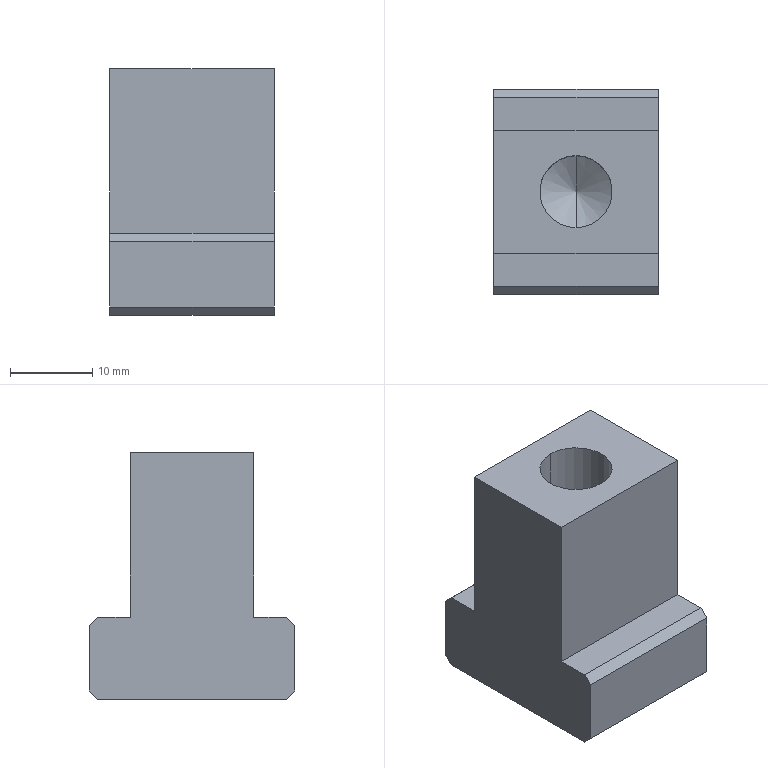Component | SolidWorks | 19-1 | 1 solid | 18 faces | box 20 x 25 x 30 mm | volume 9386 mm3 | plane 14 | cylinder 2 | cone 2 | commonest cylinder face diameters 8.8 x2
build123d program:
from build123d import *

# Parameters (mm, degrees)
SKETCH1_W                   = 20
SKETCH1_H                   = 25
EXTRUDE1_DEPTH              = 10
SKETCH2_W                   = 20
SKETCH2_H                   = 15
EXTRUDE2_DEPTH              = 20
M10X1_25_TAPPED_HOLE1_D     = 8.8
M10X1_25_TAPPED_HOLE1_DEPTH = 25
M10X1_25_TAPPED_HOLE1_TIP   = 2.644
CHAMFER1_SIZE               = 1


with BuildPart() as part:
    # Sketch1 → Extrude1 (new body)
    with BuildSketch(Plane(origin=(0, 0, 0), x_dir=(1, 0, 0), z_dir=(0, 1, 0))):
        Rectangle(SKETCH1_W, SKETCH1_H)
    extrude(amount=EXTRUDE1_DEPTH)

    # Sketch2 → Extrude2 (add)
    with BuildSketch(Plane(origin=(0, 10, 0), x_dir=(1, 0, 0), z_dir=(0, 1, 0))):
        Rectangle(SKETCH2_W, SKETCH2_H)
    extrude(amount=EXTRUDE2_DEPTH)

    # M10x1.25 Tapped Hole1
    with Locations(Plane(origin=(0, 30, 0), x_dir=(1, 0, 0), z_dir=(0, 1, 0))):
        with Locations((0, 0)):
            Hole(M10X1_25_TAPPED_HOLE1_D / 2, depth=M10X1_25_TAPPED_HOLE1_DEPTH)
            with Locations((0, 0, -(M10X1_25_TAPPED_HOLE1_DEPTH + M10X1_25_TAPPED_HOLE1_TIP / 2))):  # 118° drill point
                Cone(0, M10X1_25_TAPPED_HOLE1_D / 2, M10X1_25_TAPPED_HOLE1_TIP, mode=Mode.SUBTRACT)

    # Chamfer1
    chamfer1_edges = [part.edges().sort_by_distance(p)[0] for p in [
        (0, 10, -12.5),
        (0, 0, -12.5),
        (0, 10, 12.5),
        (0, 0, 12.5),
    ]]
    chamfer(chamfer1_edges, length=CHAMFER1_SIZE)


solid = part.part

# Placed as in the assembly
solid = solid.moved(Location((-102.5, -29.5, 100.8), (90, 0, 0)))
STEP:
#1=COLOUR_RGB('',0.7922,0.8196,0.9333);
#2=FILL_AREA_STYLE_COLOUR('',#1);
#3=FILL_AREA_STYLE('',(#2));
#4=SURFACE_STYLE_FILL_AREA(#3);
#5=SURFACE_SIDE_STYLE('',(#4));
#6=SURFACE_STYLE_USAGE(.BOTH.,#5);
#7=PRESENTATION_STYLE_ASSIGNMENT((#6));
#8=CARTESIAN_POINT('',(-4.035,-0.9882,4.165));
#9=VERTEX_POINT('',#8);
#10=CARTESIAN_POINT('',(-4.035,-1.335,4.165));
#11=VERTEX_POINT('',#10);
#12=CARTESIAN_POINT('',(-4.035,-1.161,4.165));
#13=DIRECTION('',(0.,0.,1.));
#14=DIRECTION('',(0.,-1.,0.));
#15=AXIS2_PLACEMENT_3D('',#12,#13,#14);
#16=CIRCLE('',#15,0.1732);
#17=EDGE_CURVE('',#9,#11,#16,.T.);
#18=ORIENTED_EDGE('',*,*,#17,.F.);
#19=CARTESIAN_POINT('',(-4.035,-0.9882,5.15));
#20=VERTEX_POINT('',#19);
#21=CARTESIAN_POINT('',(-4.035,-0.9882,5.15));
#22=DIRECTION('',(0.,0.,1.));
#23=VECTOR('',#22,39.37);
#24=LINE('',#21,#23);
#25=EDGE_CURVE('',#9,#20,#24,.T.);
#26=ORIENTED_EDGE('',*,*,#25,.T.);
#27=CARTESIAN_POINT('',(-4.035,-1.335,5.15));
#28=VERTEX_POINT('',#27);
#29=CARTESIAN_POINT('',(-4.035,-1.161,5.15));
#30=DIRECTION('',(0.,0.,1.));
#31=DIRECTION('',(0.,-1.,0.));
#32=AXIS2_PLACEMENT_3D('',#29,#30,#31);
#33=CIRCLE('',#32,0.1732);
#34=EDGE_CURVE('',#20,#28,#33,.T.);
#35=ORIENTED_EDGE('',*,*,#34,.T.);
#36=CARTESIAN_POINT('',(-4.035,-1.335,5.15));
#37=DIRECTION('',(0.,0.,1.));
#38=VECTOR('',#37,39.37);
#39=LINE('',#36,#38);
#40=EDGE_CURVE('',#11,#28,#39,.T.);
#41=ORIENTED_EDGE('',*,*,#40,.F.);
#42=EDGE_LOOP('',(#18,#26,#35,#41));
#43=FACE_OUTER_BOUND('',#42,.T.);
#44=CARTESIAN_POINT('',(-4.035,-1.161,5.15));
#45=DIRECTION('',(0.,0.,1.));
#46=DIRECTION('',(0.,-1.,0.));
#47=AXIS2_PLACEMENT_3D('',#44,#45,#46);
#48=CYLINDRICAL_SURFACE('',#47,0.1732);
#49=ADVANCED_FACE('',(#43),#48,.F.);
#50=CARTESIAN_POINT('',(-4.035,-1.161,4.061));
#51=VERTEX_POINT('',#50);
#52=CARTESIAN_POINT('',(-4.035,-1.335,4.165));
#53=DIRECTION('',(0.,-0.8572,0.515));
#54=VECTOR('',#53,39.37);
#55=LINE('',#52,#54);
#56=EDGE_CURVE('',#51,#11,#55,.T.);
#57=ORIENTED_EDGE('',*,*,#56,.F.);
#58=CARTESIAN_POINT('',(-4.035,-0.9882,4.165));
#59=DIRECTION('',(0.,0.8572,0.515));
#60=VECTOR('',#59,39.37);
#61=LINE('',#58,#60);
#62=EDGE_CURVE('',#51,#9,#61,.T.);
#63=ORIENTED_EDGE('',*,*,#62,.T.);
#64=ORIENTED_EDGE('',*,*,#17,.T.);
#65=EDGE_LOOP('',(#57,#63,#64));
#66=FACE_OUTER_BOUND('',#65,.T.);
#67=CARTESIAN_POINT('',(-4.035,-1.161,4.165));
#68=DIRECTION('',(0.,0.,1.));
#69=DIRECTION('',(0.,-1.,0.));
#70=AXIS2_PLACEMENT_3D('',#67,#68,#69);
#71=CONICAL_SURFACE('',#70,0.1732,1.03);
#72=ADVANCED_FACE('',(#66),#71,.F.);
#73=CARTESIAN_POINT('',(-3.642,-0.8661,4.362));
#74=VERTEX_POINT('',#73);
#75=CARTESIAN_POINT('',(-3.642,-0.7087,4.362));
#76=VERTEX_POINT('',#75);
#77=CARTESIAN_POINT('',(-3.642,-0.6693,4.362));
#78=DIRECTION('',(-0.,1.,-0.));
#79=VECTOR('',#78,39.37);
#80=LINE('',#77,#79);
#81=EDGE_CURVE('',#74,#76,#80,.T.);
#82=ORIENTED_EDGE('',*,*,#81,.T.);
#83=CARTESIAN_POINT('',(-4.429,-0.7087,4.362));
#84=VERTEX_POINT('',#83);
#85=CARTESIAN_POINT('',(-4.429,-0.7087,4.362));
#86=DIRECTION('',(-1.,0.,0.));
#87=VECTOR('',#86,39.37);
#88=LINE('',#85,#87);
#89=EDGE_CURVE('',#76,#84,#88,.T.);
#90=ORIENTED_EDGE('',*,*,#89,.T.);
#91=CARTESIAN_POINT('',(-4.429,-0.8661,4.362));
#92=VERTEX_POINT('',#91);
#93=CARTESIAN_POINT('',(-4.429,-0.6693,4.362));
#94=DIRECTION('',(0.,-1.,0.));
#95=VECTOR('',#94,39.37);
#96=LINE('',#93,#95);
#97=EDGE_CURVE('',#84,#92,#96,.T.);
#98=ORIENTED_EDGE('',*,*,#97,.T.);
#99=CARTESIAN_POINT('',(-4.429,-0.8661,4.362));
#100=DIRECTION('',(-1.,0.,0.));
#101=VECTOR('',#100,39.37);
#102=LINE('',#99,#101);
#103=EDGE_CURVE('',#74,#92,#102,.T.);
#104=ORIENTED_EDGE('',*,*,#103,.F.);
#105=EDGE_LOOP('',(#82,#90,#98,#104));
#106=FACE_OUTER_BOUND('',#105,.T.);
#107=CARTESIAN_POINT('',(-4.035,-1.161,4.362));
#108=DIRECTION('',(0.,0.,1.));
#109=DIRECTION('',(0.,-1.,0.));
#110=AXIS2_PLACEMENT_3D('',#107,#108,#109);
#111=PLANE('',#110);
#112=ADVANCED_FACE('',(#106),#111,.T.);
#113=ORIENTED_EDGE('',*,*,#97,.F.);
#114=CARTESIAN_POINT('',(-4.429,-0.6693,4.323));
#115=VERTEX_POINT('',#114);
#116=CARTESIAN_POINT('',(-4.429,-0.7087,4.362));
#117=DIRECTION('',(-0.,0.7071,-0.7071));
#118=VECTOR('',#117,39.37);
#119=LINE('',#116,#118);
#120=EDGE_CURVE('',#84,#115,#119,.T.);
#121=ORIENTED_EDGE('',*,*,#120,.T.);
#122=CARTESIAN_POINT('',(-4.429,-0.6693,4.008));
#123=VERTEX_POINT('',#122);
#124=CARTESIAN_POINT('',(-4.429,-0.6693,4.362));
#125=DIRECTION('',(-0.,-0.,-1.));
#126=VECTOR('',#125,39.37);
#127=LINE('',#124,#126);
#128=EDGE_CURVE('',#115,#123,#127,.T.);
#129=ORIENTED_EDGE('',*,*,#128,.T.);
#130=CARTESIAN_POINT('',(-4.429,-0.7087,3.969));
#131=VERTEX_POINT('',#130);
#132=CARTESIAN_POINT('',(-4.429,-0.6693,4.008));
#133=DIRECTION('',(-0.,-0.7071,-0.7071));
#134=VECTOR('',#133,39.37);
#135=LINE('',#132,#134);
#136=EDGE_CURVE('',#123,#131,#135,.T.);
#137=ORIENTED_EDGE('',*,*,#136,.T.);
#138=CARTESIAN_POINT('',(-4.429,-1.614,3.969));
#139=VERTEX_POINT('',#138);
#140=CARTESIAN_POINT('',(-4.429,-0.6693,3.969));
#141=DIRECTION('',(0.,-1.,0.));
#142=VECTOR('',#141,39.37);
#143=LINE('',#140,#142);
#144=EDGE_CURVE('',#131,#139,#143,.T.);
#145=ORIENTED_EDGE('',*,*,#144,.T.);
#146=CARTESIAN_POINT('',(-4.429,-1.654,4.008));
#147=VERTEX_POINT('',#146);
#148=CARTESIAN_POINT('',(-4.429,-1.654,4.008));
#149=DIRECTION('',(0.,-0.7071,0.7071));
#150=VECTOR('',#149,39.37);
#151=LINE('',#148,#150);
#152=EDGE_CURVE('',#139,#147,#151,.T.);
#153=ORIENTED_EDGE('',*,*,#152,.T.);
#154=CARTESIAN_POINT('',(-4.429,-1.654,4.323));
#155=VERTEX_POINT('',#154);
#156=CARTESIAN_POINT('',(-4.429,-1.654,4.362));
#157=DIRECTION('',(-0.,-0.,-1.));
#158=VECTOR('',#157,39.37);
#159=LINE('',#156,#158);
#160=EDGE_CURVE('',#155,#147,#159,.T.);
#161=ORIENTED_EDGE('',*,*,#160,.F.);
#162=CARTESIAN_POINT('',(-4.429,-1.614,4.362));
#163=VERTEX_POINT('',#162);
#164=CARTESIAN_POINT('',(-4.429,-1.614,4.362));
#165=DIRECTION('',(0.,0.7071,0.7071));
#166=VECTOR('',#165,39.37);
#167=LINE('',#164,#166);
#168=EDGE_CURVE('',#155,#163,#167,.T.);
#169=ORIENTED_EDGE('',*,*,#168,.T.);
#170=CARTESIAN_POINT('',(-4.429,-1.457,4.362));
#171=VERTEX_POINT('',#170);
#172=CARTESIAN_POINT('',(-4.429,-0.6693,4.362));
#173=DIRECTION('',(0.,-1.,0.));
#174=VECTOR('',#173,39.37);
#175=LINE('',#172,#174);
#176=EDGE_CURVE('',#171,#163,#175,.T.);
#177=ORIENTED_EDGE('',*,*,#176,.F.);
#178=CARTESIAN_POINT('',(-4.429,-1.457,5.15));
#179=VERTEX_POINT('',#178);
#180=CARTESIAN_POINT('',(-4.429,-1.457,5.15));
#181=DIRECTION('',(-0.,-0.,-1.));
#182=VECTOR('',#181,39.37);
#183=LINE('',#180,#182);
#184=EDGE_CURVE('',#179,#171,#183,.T.);
#185=ORIENTED_EDGE('',*,*,#184,.F.);
#186=CARTESIAN_POINT('',(-4.429,-0.8661,5.15));
#187=VERTEX_POINT('',#186);
#188=CARTESIAN_POINT('',(-4.429,-0.8661,5.15));
#189=DIRECTION('',(-0.,-1.,0.));
#190=VECTOR('',#189,39.37);
#191=LINE('',#188,#190);
#192=EDGE_CURVE('',#187,#179,#191,.T.);
#193=ORIENTED_EDGE('',*,*,#192,.F.);
#194=CARTESIAN_POINT('',(-4.429,-0.8661,5.15));
#195=DIRECTION('',(-0.,-0.,-1.));
#196=VECTOR('',#195,39.37);
#197=LINE('',#194,#196);
#198=EDGE_CURVE('',#187,#92,#197,.T.);
#199=ORIENTED_EDGE('',*,*,#198,.T.);
#200=EDGE_LOOP('',(#113,#121,#129,#137,#145,#153,#161,#169,#177,#185,#193,#199));
#201=FACE_OUTER_BOUND('',#200,.T.);
#202=CARTESIAN_POINT('',(-4.429,-0.6693,4.362));
#203=DIRECTION('',(1.,-0.,-0.));
#204=DIRECTION('',(-0.,1.,-0.));
#205=AXIS2_PLACEMENT_3D('',#202,#203,#204);
#206=PLANE('',#205);
#207=ADVANCED_FACE('',(#201),#206,.F.);
#208=CARTESIAN_POINT('',(-3.642,-1.654,4.323));
#209=VERTEX_POINT('',#208);
#210=CARTESIAN_POINT('',(-3.642,-1.654,4.008));
#211=VERTEX_POINT('',#210);
#212=CARTESIAN_POINT('',(-3.642,-1.654,4.362));
#213=DIRECTION('',(-0.,-0.,-1.));
#214=VECTOR('',#213,39.37);
#215=LINE('',#212,#214);
#216=EDGE_CURVE('',#209,#211,#215,.T.);
#217=ORIENTED_EDGE('',*,*,#216,.F.);
#218=CARTESIAN_POINT('',(-4.429,-1.654,4.323));
#219=DIRECTION('',(-1.,0.,0.));
#220=VECTOR('',#219,39.37);
#221=LINE('',#218,#220);
#222=EDGE_CURVE('',#209,#155,#221,.T.);
#223=ORIENTED_EDGE('',*,*,#222,.T.);
#224=ORIENTED_EDGE('',*,*,#160,.T.);
#225=CARTESIAN_POINT('',(-4.429,-1.654,4.008));
#226=DIRECTION('',(1.,-0.,-0.));
#227=VECTOR('',#226,39.37);
#228=LINE('',#225,#227);
#229=EDGE_CURVE('',#147,#211,#228,.T.);
#230=ORIENTED_EDGE('',*,*,#229,.T.);
#231=EDGE_LOOP('',(#217,#223,#224,#230));
#232=FACE_OUTER_BOUND('',#231,.T.);
#233=CARTESIAN_POINT('',(-4.429,-1.654,4.362));
#234=DIRECTION('',(0.,1.,-0.));
#235=DIRECTION('',(-1.,0.,0.));
#236=AXIS2_PLACEMENT_3D('',#233,#234,#235);
#237=PLANE('',#236);
#238=ADVANCED_FACE('',(#232),#237,.F.);
#239=CARTESIAN_POINT('',(-3.642,-0.6693,4.323));
#240=VERTEX_POINT('',#239);
#241=CARTESIAN_POINT('',(-3.642,-0.6693,4.008));
#242=VERTEX_POINT('',#241);
#243=CARTESIAN_POINT('',(-3.642,-0.6693,4.362));
#244=DIRECTION('',(-0.,-0.,-1.));
#245=VECTOR('',#244,39.37);
#246=LINE('',#243,#245);
#247=EDGE_CURVE('',#240,#242,#246,.T.);
#248=ORIENTED_EDGE('',*,*,#247,.F.);
#249=CARTESIAN_POINT('',(-3.642,-0.7087,4.362));
#250=DIRECTION('',(0.,-0.7071,0.7071));
#251=VECTOR('',#250,39.37);
#252=LINE('',#249,#251);
#253=EDGE_CURVE('',#240,#76,#252,.T.);
#254=ORIENTED_EDGE('',*,*,#253,.T.);
#255=ORIENTED_EDGE('',*,*,#81,.F.);
#256=CARTESIAN_POINT('',(-3.642,-0.8661,5.15));
#257=VERTEX_POINT('',#256);
#258=CARTESIAN_POINT('',(-3.642,-0.8661,5.15));
#259=DIRECTION('',(-0.,-0.,-1.));
#260=VECTOR('',#259,39.37);
#261=LINE('',#258,#260);
#262=EDGE_CURVE('',#257,#74,#261,.T.);
#263=ORIENTED_EDGE('',*,*,#262,.F.);
#264=CARTESIAN_POINT('',(-3.642,-1.457,5.15));
#265=VERTEX_POINT('',#264);
#266=CARTESIAN_POINT('',(-3.642,-0.8661,5.15));
#267=DIRECTION('',(-0.,1.,-0.));
#268=VECTOR('',#267,39.37);
#269=LINE('',#266,#268);
#270=EDGE_CURVE('',#265,#257,#269,.T.);
#271=ORIENTED_EDGE('',*,*,#270,.F.);
#272=CARTESIAN_POINT('',(-3.642,-1.457,4.362));
#273=VERTEX_POINT('',#272);
#274=CARTESIAN_POINT('',(-3.642,-1.457,5.15));
#275=DIRECTION('',(-0.,-0.,-1.));
#276=VECTOR('',#275,39.37);
#277=LINE('',#274,#276);
#278=EDGE_CURVE('',#265,#273,#277,.T.);
#279=ORIENTED_EDGE('',*,*,#278,.T.);
#280=CARTESIAN_POINT('',(-3.642,-1.614,4.362));
#281=VERTEX_POINT('',#280);
#282=CARTESIAN_POINT('',(-3.642,-0.6693,4.362));
#283=DIRECTION('',(-0.,1.,-0.));
#284=VECTOR('',#283,39.37);
#285=LINE('',#282,#284);
#286=EDGE_CURVE('',#281,#273,#285,.T.);
#287=ORIENTED_EDGE('',*,*,#286,.F.);
#288=CARTESIAN_POINT('',(-3.642,-1.614,4.362));
#289=DIRECTION('',(-0.,-0.7071,-0.7071));
#290=VECTOR('',#289,39.37);
#291=LINE('',#288,#290);
#292=EDGE_CURVE('',#281,#209,#291,.T.);
#293=ORIENTED_EDGE('',*,*,#292,.T.);
#294=ORIENTED_EDGE('',*,*,#216,.T.);
#295=CARTESIAN_POINT('',(-3.642,-1.614,3.969));
#296=VERTEX_POINT('',#295);
#297=CARTESIAN_POINT('',(-3.642,-1.654,4.008));
#298=DIRECTION('',(-0.,0.7071,-0.7071));
#299=VECTOR('',#298,39.37);
#300=LINE('',#297,#299);
#301=EDGE_CURVE('',#211,#296,#300,.T.);
#302=ORIENTED_EDGE('',*,*,#301,.T.);
#303=CARTESIAN_POINT('',(-3.642,-0.7087,3.969));
#304=VERTEX_POINT('',#303);
#305=CARTESIAN_POINT('',(-3.642,-0.6693,3.969));
#306=DIRECTION('',(-0.,1.,-0.));
#307=VECTOR('',#306,39.37);
#308=LINE('',#305,#307);
#309=EDGE_CURVE('',#296,#304,#308,.T.);
#310=ORIENTED_EDGE('',*,*,#309,.T.);
#311=CARTESIAN_POINT('',(-3.642,-0.6693,4.008));
#312=DIRECTION('',(0.,0.7071,0.7071));
#313=VECTOR('',#312,39.37);
#314=LINE('',#311,#313);
#315=EDGE_CURVE('',#304,#242,#314,.T.);
#316=ORIENTED_EDGE('',*,*,#315,.T.);
#317=EDGE_LOOP('',(#248,#254,#255,#263,#271,#279,#287,#293,#294,#302,#310,#316));
#318=FACE_OUTER_BOUND('',#317,.T.);
#319=CARTESIAN_POINT('',(-3.642,-0.6693,4.362));
#320=DIRECTION('',(-1.,0.,0.));
#321=DIRECTION('',(0.,-1.,0.));
#322=AXIS2_PLACEMENT_3D('',#319,#320,#321);
#323=PLANE('',#322);
#324=ADVANCED_FACE('',(#318),#323,.F.);
#325=ORIENTED_EDGE('',*,*,#128,.F.);
#326=CARTESIAN_POINT('',(-3.642,-0.6693,4.323));
#327=DIRECTION('',(1.,-0.,-0.));
#328=VECTOR('',#327,39.37);
#329=LINE('',#326,#328);
#330=EDGE_CURVE('',#115,#240,#329,.T.);
#331=ORIENTED_EDGE('',*,*,#330,.T.);
#332=ORIENTED_EDGE('',*,*,#247,.T.);
#333=CARTESIAN_POINT('',(-4.429,-0.6693,4.008));
#334=DIRECTION('',(-1.,0.,0.));
#335=VECTOR('',#334,39.37);
#336=LINE('',#333,#335);
#337=EDGE_CURVE('',#242,#123,#336,.T.);
#338=ORIENTED_EDGE('',*,*,#337,.T.);
#339=EDGE_LOOP('',(#325,#331,#332,#338));
#340=FACE_OUTER_BOUND('',#339,.T.);
#341=CARTESIAN_POINT('',(-4.429,-0.6693,4.362));
#342=DIRECTION('',(-0.,-1.,0.));
#343=DIRECTION('',(1.,-0.,-0.));
#344=AXIS2_PLACEMENT_3D('',#341,#342,#343);
#345=PLANE('',#344);
#346=ADVANCED_FACE('',(#340),#345,.F.);
#347=ORIENTED_EDGE('',*,*,#176,.T.);
#348=CARTESIAN_POINT('',(-3.642,-1.614,4.362));
#349=DIRECTION('',(1.,-0.,-0.));
#350=VECTOR('',#349,39.37);
#351=LINE('',#348,#350);
#352=EDGE_CURVE('',#163,#281,#351,.T.);
#353=ORIENTED_EDGE('',*,*,#352,.T.);
#354=ORIENTED_EDGE('',*,*,#286,.T.);
#355=CARTESIAN_POINT('',(-4.429,-1.457,4.362));
#356=DIRECTION('',(1.,-0.,-0.));
#357=VECTOR('',#356,39.37);
#358=LINE('',#355,#357);
#359=EDGE_CURVE('',#171,#273,#358,.T.);
#360=ORIENTED_EDGE('',*,*,#359,.F.);
#361=EDGE_LOOP('',(#347,#353,#354,#360));
#362=FACE_OUTER_BOUND('',#361,.T.);
#363=CARTESIAN_POINT('',(-4.035,-1.161,4.362));
#364=DIRECTION('',(0.,0.,1.));
#365=DIRECTION('',(0.,-1.,0.));
#366=AXIS2_PLACEMENT_3D('',#363,#364,#365);
#367=PLANE('',#366);
#368=ADVANCED_FACE('',(#362),#367,.T.);
#369=ORIENTED_EDGE('',*,*,#144,.F.);
#370=CARTESIAN_POINT('',(-4.035,-0.7087,3.969));
#371=DIRECTION('',(1.,-0.,-0.));
#372=VECTOR('',#371,39.37);
#373=LINE('',#370,#372);
#374=EDGE_CURVE('',#131,#304,#373,.T.);
#375=ORIENTED_EDGE('',*,*,#374,.T.);
#376=ORIENTED_EDGE('',*,*,#309,.F.);
#377=CARTESIAN_POINT('',(-4.035,-1.614,3.969));
#378=DIRECTION('',(-1.,0.,0.));
#379=VECTOR('',#378,39.37);
#380=LINE('',#377,#379);
#381=EDGE_CURVE('',#296,#139,#380,.T.);
#382=ORIENTED_EDGE('',*,*,#381,.T.);
#383=EDGE_LOOP('',(#369,#375,#376,#382));
#384=FACE_OUTER_BOUND('',#383,.T.);
#385=CARTESIAN_POINT('',(-4.035,-1.161,3.969));
#386=DIRECTION('',(0.,0.,1.));
#387=DIRECTION('',(0.,-1.,0.));
#388=AXIS2_PLACEMENT_3D('',#385,#386,#387);
#389=PLANE('',#388);
#390=ADVANCED_FACE('',(#384),#389,.F.);
#391=ORIENTED_EDGE('',*,*,#359,.T.);
#392=ORIENTED_EDGE('',*,*,#278,.F.);
#393=CARTESIAN_POINT('',(-4.429,-1.457,5.15));
#394=DIRECTION('',(1.,-0.,-0.));
#395=VECTOR('',#394,39.37);
#396=LINE('',#393,#395);
#397=EDGE_CURVE('',#179,#265,#396,.T.);
#398=ORIENTED_EDGE('',*,*,#397,.F.);
#399=ORIENTED_EDGE('',*,*,#184,.T.);
#400=EDGE_LOOP('',(#391,#392,#398,#399));
#401=FACE_OUTER_BOUND('',#400,.T.);
#402=CARTESIAN_POINT('',(-4.429,-1.457,5.15));
#403=DIRECTION('',(0.,1.,-0.));
#404=DIRECTION('',(-1.,0.,0.));
#405=AXIS2_PLACEMENT_3D('',#402,#403,#404);
#406=PLANE('',#405);
#407=ADVANCED_FACE('',(#401),#406,.F.);
#408=ORIENTED_EDGE('',*,*,#103,.T.);
#409=ORIENTED_EDGE('',*,*,#198,.F.);
#410=CARTESIAN_POINT('',(-4.429,-0.8661,5.15));
#411=DIRECTION('',(-1.,0.,0.));
#412=VECTOR('',#411,39.37);
#413=LINE('',#410,#412);
#414=EDGE_CURVE('',#257,#187,#413,.T.);
#415=ORIENTED_EDGE('',*,*,#414,.F.);
#416=ORIENTED_EDGE('',*,*,#262,.T.);
#417=EDGE_LOOP('',(#408,#409,#415,#416));
#418=FACE_OUTER_BOUND('',#417,.T.);
#419=CARTESIAN_POINT('',(-4.429,-0.8661,5.15));
#420=DIRECTION('',(-0.,-1.,0.));
#421=DIRECTION('',(1.,-0.,-0.));
#422=AXIS2_PLACEMENT_3D('',#419,#420,#421);
#423=PLANE('',#422);
#424=ADVANCED_FACE('',(#418),#423,.F.);
#425=CARTESIAN_POINT('',(-4.035,-1.161,5.15));
#426=DIRECTION('',(0.,0.,1.));
#427=DIRECTION('',(0.,-1.,0.));
#428=AXIS2_PLACEMENT_3D('',#425,#426,#427);
#429=CIRCLE('',#428,0.1732);
#430=EDGE_CURVE('',#28,#20,#429,.T.);
#431=ORIENTED_EDGE('',*,*,#430,.F.);
#432=ORIENTED_EDGE('',*,*,#34,.F.);
#433=EDGE_LOOP('',(#431,#432));
#434=FACE_BOUND('',#433,.T.);
#435=ORIENTED_EDGE('',*,*,#192,.T.);
#436=ORIENTED_EDGE('',*,*,#397,.T.);
#437=ORIENTED_EDGE('',*,*,#270,.T.);
#438=ORIENTED_EDGE('',*,*,#414,.T.);
#439=EDGE_LOOP('',(#435,#436,#437,#438));
#440=FACE_OUTER_BOUND('',#439,.T.);
#441=CARTESIAN_POINT('',(-4.035,-1.161,5.15));
#442=DIRECTION('',(0.,0.,1.));
#443=DIRECTION('',(0.,-1.,0.));
#444=AXIS2_PLACEMENT_3D('',#441,#442,#443);
#445=PLANE('',#444);
#446=ADVANCED_FACE('',(#434,#440),#445,.T.);
#447=ORIENTED_EDGE('',*,*,#62,.F.);
#448=ORIENTED_EDGE('',*,*,#56,.T.);
#449=CARTESIAN_POINT('',(-4.035,-1.161,4.165));
#450=DIRECTION('',(0.,0.,1.));
#451=DIRECTION('',(0.,-1.,0.));
#452=AXIS2_PLACEMENT_3D('',#449,#450,#451);
#453=CIRCLE('',#452,0.1732);
#454=EDGE_CURVE('',#11,#9,#453,.T.);
#455=ORIENTED_EDGE('',*,*,#454,.T.);
#456=EDGE_LOOP('',(#447,#448,#455));
#457=FACE_OUTER_BOUND('',#456,.T.);
#458=CARTESIAN_POINT('',(-4.035,-1.161,4.165));
#459=DIRECTION('',(0.,0.,1.));
#460=DIRECTION('',(0.,-1.,0.));
#461=AXIS2_PLACEMENT_3D('',#458,#459,#460);
#462=CONICAL_SURFACE('',#461,0.1732,1.03);
#463=ADVANCED_FACE('',(#457),#462,.F.);
#464=ORIENTED_EDGE('',*,*,#25,.F.);
#465=ORIENTED_EDGE('',*,*,#454,.F.);
#466=ORIENTED_EDGE('',*,*,#40,.T.);
#467=ORIENTED_EDGE('',*,*,#430,.T.);
#468=EDGE_LOOP('',(#464,#465,#466,#467));
#469=FACE_OUTER_BOUND('',#468,.T.);
#470=CARTESIAN_POINT('',(-4.035,-1.161,5.15));
#471=DIRECTION('',(0.,0.,1.));
#472=DIRECTION('',(0.,-1.,0.));
#473=AXIS2_PLACEMENT_3D('',#470,#471,#472);
#474=CYLINDRICAL_SURFACE('',#473,0.1732);
#475=ADVANCED_FACE('',(#469),#474,.F.);
#476=ORIENTED_EDGE('',*,*,#253,.F.);
#477=ORIENTED_EDGE('',*,*,#330,.F.);
#478=ORIENTED_EDGE('',*,*,#120,.F.);
#479=ORIENTED_EDGE('',*,*,#89,.F.);
#480=EDGE_LOOP('',(#476,#477,#478,#479));
#481=FACE_OUTER_BOUND('',#480,.T.);
#482=CARTESIAN_POINT('',(-4.035,-0.7087,4.362));
#483=DIRECTION('',(0.,0.7071,0.7071));
#484=DIRECTION('',(1.,-0.,-0.));
#485=AXIS2_PLACEMENT_3D('',#482,#483,#484);
#486=PLANE('',#485);
#487=ADVANCED_FACE('',(#481),#486,.T.);
#488=ORIENTED_EDGE('',*,*,#315,.F.);
#489=ORIENTED_EDGE('',*,*,#374,.F.);
#490=ORIENTED_EDGE('',*,*,#136,.F.);
#491=ORIENTED_EDGE('',*,*,#337,.F.);
#492=EDGE_LOOP('',(#488,#489,#490,#491));
#493=FACE_OUTER_BOUND('',#492,.T.);
#494=CARTESIAN_POINT('',(-4.429,-0.6693,4.008));
#495=DIRECTION('',(0.,-0.7071,0.7071));
#496=DIRECTION('',(-1.,0.,0.));
#497=AXIS2_PLACEMENT_3D('',#494,#495,#496);
#498=PLANE('',#497);
#499=ADVANCED_FACE('',(#493),#498,.F.);
#500=ORIENTED_EDGE('',*,*,#168,.F.);
#501=ORIENTED_EDGE('',*,*,#222,.F.);
#502=ORIENTED_EDGE('',*,*,#292,.F.);
#503=ORIENTED_EDGE('',*,*,#352,.F.);
#504=EDGE_LOOP('',(#500,#501,#502,#503));
#505=FACE_OUTER_BOUND('',#504,.T.);
#506=CARTESIAN_POINT('',(-4.035,-1.614,4.362));
#507=DIRECTION('',(0.,-0.7071,0.7071));
#508=DIRECTION('',(-1.,0.,0.));
#509=AXIS2_PLACEMENT_3D('',#506,#507,#508);
#510=PLANE('',#509);
#511=ADVANCED_FACE('',(#505),#510,.T.);
#512=ORIENTED_EDGE('',*,*,#152,.F.);
#513=ORIENTED_EDGE('',*,*,#381,.F.);
#514=ORIENTED_EDGE('',*,*,#301,.F.);
#515=ORIENTED_EDGE('',*,*,#229,.F.);
#516=EDGE_LOOP('',(#512,#513,#514,#515));
#517=FACE_OUTER_BOUND('',#516,.T.);
#518=CARTESIAN_POINT('',(-4.429,-1.654,4.008));
#519=DIRECTION('',(0.,0.7071,0.7071));
#520=DIRECTION('',(1.,-0.,-0.));
#521=AXIS2_PLACEMENT_3D('',#518,#519,#520);
#522=PLANE('',#521);
#523=ADVANCED_FACE('',(#517),#522,.F.);
#524=CLOSED_SHELL('',(#49,#72,#112,#207,#238,#324,#346,#368,#390,#407,#424,#446,#463,#475,#487,#499,#511,#523));
#525=MANIFOLD_SOLID_BREP('',#524);
#526=STYLED_ITEM('',(#7),#525);
#527=(LENGTH_UNIT()NAMED_UNIT(*)SI_UNIT($,.METRE.));
#528=LENGTH_MEASURE_WITH_UNIT(LENGTH_MEASURE(0.0254),#527);
#529=DIMENSIONAL_EXPONENTS(1.,0.,0.,0.,0.,0.,0.);
#530=(CONVERSION_BASED_UNIT('',#528)LENGTH_UNIT()NAMED_UNIT(#529));
#531=UNCERTAINTY_MEASURE_WITH_UNIT(LENGTH_MEASURE(0.00001),#530,'','');
#532=(NAMED_UNIT(*)PLANE_ANGLE_UNIT()SI_UNIT($,.RADIAN.));
#533=(NAMED_UNIT(*)SI_UNIT($,.STERADIAN.)SOLID_ANGLE_UNIT());
#534=(GEOMETRIC_REPRESENTATION_CONTEXT(3)GLOBAL_UNCERTAINTY_ASSIGNED_CONTEXT((#531))GLOBAL_UNIT_ASSIGNED_CONTEXT((#530,#532,#533))REPRESENTATION_CONTEXT('',''));
#535=MECHANICAL_DESIGN_GEOMETRIC_PRESENTATION_REPRESENTATION('',(#526),#534);
#536=PRESENTATION_LAYER_ASSIGNMENT('','',(#526));
#537=CARTESIAN_POINT('',(0.,0.,0.));
#538=DIRECTION('',(0.,0.,1.));
#539=DIRECTION('',(1.,0.,0.));
#540=AXIS2_PLACEMENT_3D('',#537,#538,#539);
#541=(LENGTH_UNIT()NAMED_UNIT(*)SI_UNIT($,.METRE.));
#542=LENGTH_MEASURE_WITH_UNIT(LENGTH_MEASURE(0.0254),#541);
#543=DIMENSIONAL_EXPONENTS(1.,0.,0.,0.,0.,0.,0.);
#544=(CONVERSION_BASED_UNIT('',#542)LENGTH_UNIT()NAMED_UNIT(#543));
#545=UNCERTAINTY_MEASURE_WITH_UNIT(LENGTH_MEASURE(0.00001),#544,'','');
#546=(NAMED_UNIT(*)PLANE_ANGLE_UNIT()SI_UNIT($,.RADIAN.));
#547=(NAMED_UNIT(*)SI_UNIT($,.STERADIAN.)SOLID_ANGLE_UNIT());
#548=(GEOMETRIC_REPRESENTATION_CONTEXT(3)GLOBAL_UNCERTAINTY_ASSIGNED_CONTEXT((#545))GLOBAL_UNIT_ASSIGNED_CONTEXT((#544,#546,#547))REPRESENTATION_CONTEXT('',''));
#549=ADVANCED_BREP_SHAPE_REPRESENTATION('',(#525,#540),#548);